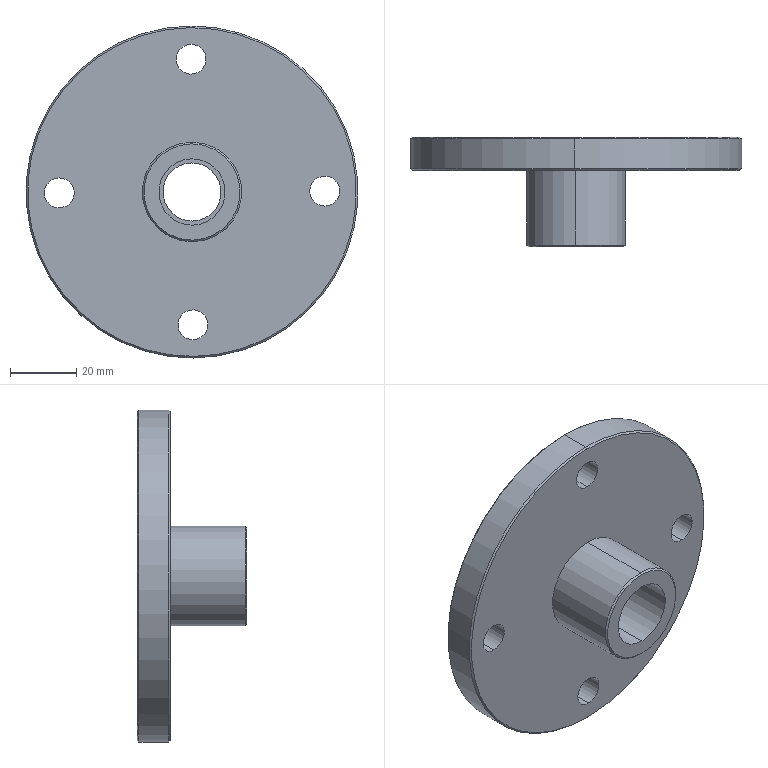Component | SolidWorks | E004Tray-1 | 1 solid | 28 faces | box 100 x 33 x 100 mm | volume 82304 mm3 | cylinder 16 | cone 8 | plane 4 | commonest cylinder face diameters 9 x8 20 x2 17.5 x2 100 x2 30 x2 | material Plain Carbon Steel
STEP:
#1=COLOUR_RGB('',0.7922,0.8196,0.9333);
#2=FILL_AREA_STYLE_COLOUR('',#1);
#3=FILL_AREA_STYLE('',(#2));
#4=SURFACE_STYLE_FILL_AREA(#3);
#5=SURFACE_SIDE_STYLE('',(#4));
#6=SURFACE_STYLE_USAGE(.BOTH.,#5);
#7=PRESENTATION_STYLE_ASSIGNMENT((#6));
#8=CARTESIAN_POINT('',(0.002756,9.764,-0.3937));
#9=VERTEX_POINT('',#8);
#10=CARTESIAN_POINT('',(-0.002756,9.764,0.3937));
#11=VERTEX_POINT('',#10);
#12=CARTESIAN_POINT('',(0.,9.764,0.));
#13=DIRECTION('',(0.,-1.,0.));
#14=DIRECTION('',(-0.006999,0.,1.));
#15=AXIS2_PLACEMENT_3D('',#12,#13,#14);
#16=CIRCLE('',#15,0.3937);
#17=EDGE_CURVE('',#9,#11,#16,.T.);
#18=ORIENTED_EDGE('',*,*,#17,.T.);
#19=CARTESIAN_POINT('',(-0.002756,10.787,0.3937));
#20=VERTEX_POINT('',#19);
#21=CARTESIAN_POINT('',(-0.002756,11.063,0.3937));
#22=DIRECTION('',(0.,1.,0.));
#23=VECTOR('',#22,39.37);
#24=LINE('',#21,#23);
#25=EDGE_CURVE('',#11,#20,#24,.T.);
#26=ORIENTED_EDGE('',*,*,#25,.T.);
#27=CARTESIAN_POINT('',(0.002756,10.787,-0.3937));
#28=VERTEX_POINT('',#27);
#29=CARTESIAN_POINT('',(0.,10.787,0.));
#30=DIRECTION('',(0.,1.,0.));
#31=DIRECTION('',(0.006999,0.,-1.));
#32=AXIS2_PLACEMENT_3D('',#29,#30,#31);
#33=CIRCLE('',#32,0.3937);
#34=EDGE_CURVE('',#20,#28,#33,.T.);
#35=ORIENTED_EDGE('',*,*,#34,.T.);
#36=CARTESIAN_POINT('',(0.002756,11.063,-0.3937));
#37=DIRECTION('',(0.,1.,0.));
#38=VECTOR('',#37,39.37);
#39=LINE('',#36,#38);
#40=EDGE_CURVE('',#9,#28,#39,.T.);
#41=ORIENTED_EDGE('',*,*,#40,.F.);
#42=EDGE_LOOP('',(#18,#26,#35,#41));
#43=FACE_OUTER_BOUND('',#42,.T.);
#44=CARTESIAN_POINT('',(0.,11.063,0.));
#45=DIRECTION('',(0.,1.,0.));
#46=DIRECTION('',(0.006999,0.,-1.));
#47=AXIS2_PLACEMENT_3D('',#44,#45,#46);
#48=CYLINDRICAL_SURFACE('',#47,0.3937);
#49=ADVANCED_FACE('',(#43),#48,.F.);
#50=CARTESIAN_POINT('',(-0.003996,9.764,0.5709));
#51=VERTEX_POINT('',#50);
#52=CARTESIAN_POINT('',(0.003996,9.764,-0.5709));
#53=VERTEX_POINT('',#52);
#54=CARTESIAN_POINT('',(0.,9.764,0.));
#55=DIRECTION('',(0.,-1.,0.));
#56=DIRECTION('',(-0.006999,0.,1.));
#57=AXIS2_PLACEMENT_3D('',#54,#55,#56);
#58=CIRCLE('',#57,0.5709);
#59=EDGE_CURVE('',#51,#53,#58,.T.);
#60=ORIENTED_EDGE('',*,*,#59,.F.);
#61=CARTESIAN_POINT('',(-0.004134,9.783,0.5905));
#62=VERTEX_POINT('',#61);
#63=CARTESIAN_POINT('',(-0.004134,9.783,0.5905));
#64=DIRECTION('',(-0.004949,0.7071,0.7071));
#65=VECTOR('',#64,39.37);
#66=LINE('',#63,#65);
#67=EDGE_CURVE('',#51,#62,#66,.T.);
#68=ORIENTED_EDGE('',*,*,#67,.T.);
#69=CARTESIAN_POINT('',(0.004134,9.783,-0.5905));
#70=VERTEX_POINT('',#69);
#71=CARTESIAN_POINT('',(0.,9.783,0.));
#72=DIRECTION('',(0.,1.,0.));
#73=DIRECTION('',(-0.006999,0.,1.));
#74=AXIS2_PLACEMENT_3D('',#71,#72,#73);
#75=CIRCLE('',#74,0.5906);
#76=EDGE_CURVE('',#70,#62,#75,.T.);
#77=ORIENTED_EDGE('',*,*,#76,.F.);
#78=CARTESIAN_POINT('',(0.004134,9.783,-0.5905));
#79=DIRECTION('',(0.004949,0.7071,-0.7071));
#80=VECTOR('',#79,39.37);
#81=LINE('',#78,#80);
#82=EDGE_CURVE('',#53,#70,#81,.T.);
#83=ORIENTED_EDGE('',*,*,#82,.F.);
#84=EDGE_LOOP('',(#60,#68,#77,#83));
#85=FACE_OUTER_BOUND('',#84,.T.);
#86=CARTESIAN_POINT('',(0.,9.783,0.));
#87=DIRECTION('',(0.,1.,0.));
#88=DIRECTION('',(0.006999,0.,-1.));
#89=AXIS2_PLACEMENT_3D('',#86,#87,#88);
#90=CONICAL_SURFACE('',#89,0.5906,0.7854);
#91=ADVANCED_FACE('',(#85),#90,.T.);
#92=CARTESIAN_POINT('',(-0.01364,10.669,1.949));
#93=VERTEX_POINT('',#92);
#94=CARTESIAN_POINT('',(0.01364,10.669,-1.949));
#95=VERTEX_POINT('',#94);
#96=CARTESIAN_POINT('',(0.,10.669,0.));
#97=DIRECTION('',(0.,-1.,0.));
#98=DIRECTION('',(-0.006999,0.,1.));
#99=AXIS2_PLACEMENT_3D('',#96,#97,#98);
#100=CIRCLE('',#99,1.949);
#101=EDGE_CURVE('',#93,#95,#100,.T.);
#102=ORIENTED_EDGE('',*,*,#101,.F.);
#103=CARTESIAN_POINT('',(-0.01378,10.689,1.968));
#104=VERTEX_POINT('',#103);
#105=CARTESIAN_POINT('',(-0.01378,10.689,1.968));
#106=DIRECTION('',(-0.004949,0.7071,0.7071));
#107=VECTOR('',#106,39.37);
#108=LINE('',#105,#107);
#109=EDGE_CURVE('',#93,#104,#108,.T.);
#110=ORIENTED_EDGE('',*,*,#109,.T.);
#111=CARTESIAN_POINT('',(0.01378,10.689,-1.968));
#112=VERTEX_POINT('',#111);
#113=CARTESIAN_POINT('',(0.,10.689,0.));
#114=DIRECTION('',(0.,1.,0.));
#115=DIRECTION('',(-0.006999,0.,1.));
#116=AXIS2_PLACEMENT_3D('',#113,#114,#115);
#117=CIRCLE('',#116,1.969);
#118=EDGE_CURVE('',#112,#104,#117,.T.);
#119=ORIENTED_EDGE('',*,*,#118,.F.);
#120=CARTESIAN_POINT('',(0.01378,10.689,-1.968));
#121=DIRECTION('',(0.004949,0.7071,-0.7071));
#122=VECTOR('',#121,39.37);
#123=LINE('',#120,#122);
#124=EDGE_CURVE('',#95,#112,#123,.T.);
#125=ORIENTED_EDGE('',*,*,#124,.F.);
#126=EDGE_LOOP('',(#102,#110,#119,#125));
#127=FACE_OUTER_BOUND('',#126,.T.);
#128=CARTESIAN_POINT('',(0.,10.689,0.));
#129=DIRECTION('',(0.,1.,0.));
#130=DIRECTION('',(0.006999,0.,-1.));
#131=AXIS2_PLACEMENT_3D('',#128,#129,#130);
#132=CONICAL_SURFACE('',#131,1.969,0.7854);
#133=ADVANCED_FACE('',(#127),#132,.T.);
#134=CARTESIAN_POINT('',(0.01364,11.063,-1.949));
#135=VERTEX_POINT('',#134);
#136=CARTESIAN_POINT('',(-0.01364,11.063,1.949));
#137=VERTEX_POINT('',#136);
#138=CARTESIAN_POINT('',(0.,11.063,0.));
#139=DIRECTION('',(0.,1.,0.));
#140=DIRECTION('',(0.006999,0.,-1.));
#141=AXIS2_PLACEMENT_3D('',#138,#139,#140);
#142=CIRCLE('',#141,1.949);
#143=EDGE_CURVE('',#135,#137,#142,.T.);
#144=ORIENTED_EDGE('',*,*,#143,.F.);
#145=CARTESIAN_POINT('',(0.01378,11.043,-1.968));
#146=VERTEX_POINT('',#145);
#147=CARTESIAN_POINT('',(0.01364,11.063,-1.949));
#148=DIRECTION('',(0.004949,-0.7071,-0.7071));
#149=VECTOR('',#148,39.37);
#150=LINE('',#147,#149);
#151=EDGE_CURVE('',#135,#146,#150,.T.);
#152=ORIENTED_EDGE('',*,*,#151,.T.);
#153=CARTESIAN_POINT('',(-0.01378,11.043,1.968));
#154=VERTEX_POINT('',#153);
#155=CARTESIAN_POINT('',(0.,11.043,0.));
#156=DIRECTION('',(0.,-1.,0.));
#157=DIRECTION('',(0.006999,0.,-1.));
#158=AXIS2_PLACEMENT_3D('',#155,#156,#157);
#159=CIRCLE('',#158,1.969);
#160=EDGE_CURVE('',#154,#146,#159,.T.);
#161=ORIENTED_EDGE('',*,*,#160,.F.);
#162=CARTESIAN_POINT('',(-0.01364,11.063,1.949));
#163=DIRECTION('',(-0.004949,-0.7071,0.7071));
#164=VECTOR('',#163,39.37);
#165=LINE('',#162,#164);
#166=EDGE_CURVE('',#137,#154,#165,.T.);
#167=ORIENTED_EDGE('',*,*,#166,.F.);
#168=EDGE_LOOP('',(#144,#152,#161,#167));
#169=FACE_OUTER_BOUND('',#168,.T.);
#170=CARTESIAN_POINT('',(0.,11.063,0.));
#171=DIRECTION('',(0.,-1.,0.));
#172=DIRECTION('',(-0.006999,0.,1.));
#173=AXIS2_PLACEMENT_3D('',#170,#171,#172);
#174=CONICAL_SURFACE('',#173,1.949,0.7854);
#175=ADVANCED_FACE('',(#169),#174,.T.);
#176=CARTESIAN_POINT('',(-0.002411,11.043,0.3445));
#177=VERTEX_POINT('',#176);
#178=CARTESIAN_POINT('',(0.002411,11.043,-0.3445));
#179=VERTEX_POINT('',#178);
#180=CARTESIAN_POINT('',(0.,11.043,0.));
#181=DIRECTION('',(0.,1.,0.));
#182=DIRECTION('',(0.006999,0.,-1.));
#183=AXIS2_PLACEMENT_3D('',#180,#181,#182);
#184=CIRCLE('',#183,0.3445);
#185=EDGE_CURVE('',#177,#179,#184,.T.);
#186=ORIENTED_EDGE('',*,*,#185,.F.);
#187=CARTESIAN_POINT('',(-0.002549,11.063,0.3642));
#188=VERTEX_POINT('',#187);
#189=CARTESIAN_POINT('',(-0.002411,11.043,0.3445));
#190=DIRECTION('',(-0.004949,0.7071,0.7071));
#191=VECTOR('',#190,39.37);
#192=LINE('',#189,#191);
#193=EDGE_CURVE('',#177,#188,#192,.T.);
#194=ORIENTED_EDGE('',*,*,#193,.T.);
#195=CARTESIAN_POINT('',(0.002549,11.063,-0.3642));
#196=VERTEX_POINT('',#195);
#197=CARTESIAN_POINT('',(0.,11.063,0.));
#198=DIRECTION('',(0.,-1.,0.));
#199=DIRECTION('',(0.006999,0.,-1.));
#200=AXIS2_PLACEMENT_3D('',#197,#198,#199);
#201=CIRCLE('',#200,0.3642);
#202=EDGE_CURVE('',#196,#188,#201,.T.);
#203=ORIENTED_EDGE('',*,*,#202,.F.);
#204=CARTESIAN_POINT('',(0.002411,11.043,-0.3445));
#205=DIRECTION('',(0.004949,0.7071,-0.7071));
#206=VECTOR('',#205,39.37);
#207=LINE('',#204,#206);
#208=EDGE_CURVE('',#179,#196,#207,.T.);
#209=ORIENTED_EDGE('',*,*,#208,.F.);
#210=EDGE_LOOP('',(#186,#194,#203,#209));
#211=FACE_OUTER_BOUND('',#210,.T.);
#212=CARTESIAN_POINT('',(0.,11.043,0.));
#213=DIRECTION('',(0.,1.,0.));
#214=DIRECTION('',(0.006999,0.,-1.));
#215=AXIS2_PLACEMENT_3D('',#212,#213,#214);
#216=CONICAL_SURFACE('',#215,0.3445,0.7854);
#217=ADVANCED_FACE('',(#211),#216,.F.);
#218=CARTESIAN_POINT('',(1.576,11.063,-0.1661));
#219=VERTEX_POINT('',#218);
#220=CARTESIAN_POINT('',(1.574,11.063,0.1882));
#221=VERTEX_POINT('',#220);
#222=CARTESIAN_POINT('',(1.575,11.063,0.01102));
#223=DIRECTION('',(0.,-1.,0.));
#224=DIRECTION('',(-1.,0.,-0.006999));
#225=AXIS2_PLACEMENT_3D('',#222,#223,#224);
#226=CIRCLE('',#225,0.1772);
#227=EDGE_CURVE('',#219,#221,#226,.T.);
#228=ORIENTED_EDGE('',*,*,#227,.F.);
#229=CARTESIAN_POINT('',(1.576,10.669,-0.1661));
#230=VERTEX_POINT('',#229);
#231=CARTESIAN_POINT('',(1.576,11.063,-0.1661));
#232=DIRECTION('',(0.,-1.,0.));
#233=VECTOR('',#232,39.37);
#234=LINE('',#231,#233);
#235=EDGE_CURVE('',#219,#230,#234,.T.);
#236=ORIENTED_EDGE('',*,*,#235,.T.);
#237=CARTESIAN_POINT('',(1.574,10.669,0.1882));
#238=VERTEX_POINT('',#237);
#239=CARTESIAN_POINT('',(1.575,10.669,0.01102));
#240=DIRECTION('',(0.,-1.,0.));
#241=DIRECTION('',(-1.,0.,-0.006999));
#242=AXIS2_PLACEMENT_3D('',#239,#240,#241);
#243=CIRCLE('',#242,0.1772);
#244=EDGE_CURVE('',#230,#238,#243,.T.);
#245=ORIENTED_EDGE('',*,*,#244,.T.);
#246=CARTESIAN_POINT('',(1.574,11.063,0.1882));
#247=DIRECTION('',(0.,-1.,0.));
#248=VECTOR('',#247,39.37);
#249=LINE('',#246,#248);
#250=EDGE_CURVE('',#221,#238,#249,.T.);
#251=ORIENTED_EDGE('',*,*,#250,.F.);
#252=EDGE_LOOP('',(#228,#236,#245,#251));
#253=FACE_OUTER_BOUND('',#252,.T.);
#254=CARTESIAN_POINT('',(1.575,11.063,0.01102));
#255=DIRECTION('',(0.,-1.,0.));
#256=DIRECTION('',(-0.006999,0.,1.));
#257=AXIS2_PLACEMENT_3D('',#254,#255,#256);
#258=CYLINDRICAL_SURFACE('',#257,0.1772);
#259=ADVANCED_FACE('',(#253),#258,.F.);
#260=CARTESIAN_POINT('',(-0.009783,11.063,1.398));
#261=VERTEX_POINT('',#260);
#262=CARTESIAN_POINT('',(-0.01226,11.063,1.752));
#263=VERTEX_POINT('',#262);
#264=CARTESIAN_POINT('',(-0.01102,11.063,1.575));
#265=DIRECTION('',(0.,-1.,0.));
#266=DIRECTION('',(0.006999,0.,-1.));
#267=AXIS2_PLACEMENT_3D('',#264,#265,#266);
#268=CIRCLE('',#267,0.1772);
#269=EDGE_CURVE('',#261,#263,#268,.T.);
#270=ORIENTED_EDGE('',*,*,#269,.F.);
#271=CARTESIAN_POINT('',(-0.009783,10.669,1.398));
#272=VERTEX_POINT('',#271);
#273=CARTESIAN_POINT('',(-0.009783,11.063,1.398));
#274=DIRECTION('',(0.,-1.,0.));
#275=VECTOR('',#274,39.37);
#276=LINE('',#273,#275);
#277=EDGE_CURVE('',#261,#272,#276,.T.);
#278=ORIENTED_EDGE('',*,*,#277,.T.);
#279=CARTESIAN_POINT('',(-0.01226,10.669,1.752));
#280=VERTEX_POINT('',#279);
#281=CARTESIAN_POINT('',(-0.01102,10.669,1.575));
#282=DIRECTION('',(0.,-1.,0.));
#283=DIRECTION('',(0.006999,0.,-1.));
#284=AXIS2_PLACEMENT_3D('',#281,#282,#283);
#285=CIRCLE('',#284,0.1772);
#286=EDGE_CURVE('',#272,#280,#285,.T.);
#287=ORIENTED_EDGE('',*,*,#286,.T.);
#288=CARTESIAN_POINT('',(-0.01226,11.063,1.752));
#289=DIRECTION('',(0.,-1.,0.));
#290=VECTOR('',#289,39.37);
#291=LINE('',#288,#290);
#292=EDGE_CURVE('',#263,#280,#291,.T.);
#293=ORIENTED_EDGE('',*,*,#292,.F.);
#294=EDGE_LOOP('',(#270,#278,#287,#293));
#295=FACE_OUTER_BOUND('',#294,.T.);
#296=CARTESIAN_POINT('',(-0.01102,11.063,1.575));
#297=DIRECTION('',(0.,-1.,0.));
#298=DIRECTION('',(-0.006999,0.,1.));
#299=AXIS2_PLACEMENT_3D('',#296,#297,#298);
#300=CYLINDRICAL_SURFACE('',#299,0.1772);
#301=ADVANCED_FACE('',(#295),#300,.F.);
#302=CARTESIAN_POINT('',(-1.574,11.063,-0.1882));
#303=VERTEX_POINT('',#302);
#304=CARTESIAN_POINT('',(-1.576,11.063,0.1661));
#305=VERTEX_POINT('',#304);
#306=CARTESIAN_POINT('',(-1.575,11.063,-0.01102));
#307=DIRECTION('',(0.,-1.,0.));
#308=DIRECTION('',(1.,0.,0.006999));
#309=AXIS2_PLACEMENT_3D('',#306,#307,#308);
#310=CIRCLE('',#309,0.1772);
#311=EDGE_CURVE('',#303,#305,#310,.T.);
#312=ORIENTED_EDGE('',*,*,#311,.F.);
#313=CARTESIAN_POINT('',(-1.574,10.669,-0.1882));
#314=VERTEX_POINT('',#313);
#315=CARTESIAN_POINT('',(-1.574,11.063,-0.1882));
#316=DIRECTION('',(0.,-1.,0.));
#317=VECTOR('',#316,39.37);
#318=LINE('',#315,#317);
#319=EDGE_CURVE('',#303,#314,#318,.T.);
#320=ORIENTED_EDGE('',*,*,#319,.T.);
#321=CARTESIAN_POINT('',(-1.576,10.669,0.1661));
#322=VERTEX_POINT('',#321);
#323=CARTESIAN_POINT('',(-1.575,10.669,-0.01102));
#324=DIRECTION('',(0.,-1.,0.));
#325=DIRECTION('',(1.,0.,0.006999));
#326=AXIS2_PLACEMENT_3D('',#323,#324,#325);
#327=CIRCLE('',#326,0.1772);
#328=EDGE_CURVE('',#314,#322,#327,.T.);
#329=ORIENTED_EDGE('',*,*,#328,.T.);
#330=CARTESIAN_POINT('',(-1.576,11.063,0.1661));
#331=DIRECTION('',(0.,-1.,0.));
#332=VECTOR('',#331,39.37);
#333=LINE('',#330,#332);
#334=EDGE_CURVE('',#305,#322,#333,.T.);
#335=ORIENTED_EDGE('',*,*,#334,.F.);
#336=EDGE_LOOP('',(#312,#320,#329,#335));
#337=FACE_OUTER_BOUND('',#336,.T.);
#338=CARTESIAN_POINT('',(-1.575,11.063,-0.01102));
#339=DIRECTION('',(0.,-1.,0.));
#340=DIRECTION('',(-0.006999,0.,1.));
#341=AXIS2_PLACEMENT_3D('',#338,#339,#340);
#342=CYLINDRICAL_SURFACE('',#341,0.1772);
#343=ADVANCED_FACE('',(#337),#342,.F.);
#344=CARTESIAN_POINT('',(0.01226,11.063,-1.752));
#345=VERTEX_POINT('',#344);
#346=CARTESIAN_POINT('',(0.009783,11.063,-1.398));
#347=VERTEX_POINT('',#346);
#348=CARTESIAN_POINT('',(0.01102,11.063,-1.575));
#349=DIRECTION('',(0.,-1.,0.));
#350=DIRECTION('',(-0.006999,0.,1.));
#351=AXIS2_PLACEMENT_3D('',#348,#349,#350);
#352=CIRCLE('',#351,0.1772);
#353=EDGE_CURVE('',#345,#347,#352,.T.);
#354=ORIENTED_EDGE('',*,*,#353,.F.);
#355=CARTESIAN_POINT('',(0.01226,10.669,-1.752));
#356=VERTEX_POINT('',#355);
#357=CARTESIAN_POINT('',(0.01226,11.063,-1.752));
#358=DIRECTION('',(0.,-1.,0.));
#359=VECTOR('',#358,39.37);
#360=LINE('',#357,#359);
#361=EDGE_CURVE('',#345,#356,#360,.T.);
#362=ORIENTED_EDGE('',*,*,#361,.T.);
#363=CARTESIAN_POINT('',(0.009783,10.669,-1.398));
#364=VERTEX_POINT('',#363);
#365=CARTESIAN_POINT('',(0.01102,10.669,-1.575));
#366=DIRECTION('',(0.,-1.,0.));
#367=DIRECTION('',(-0.006999,0.,1.));
#368=AXIS2_PLACEMENT_3D('',#365,#366,#367);
#369=CIRCLE('',#368,0.1772);
#370=EDGE_CURVE('',#356,#364,#369,.T.);
#371=ORIENTED_EDGE('',*,*,#370,.T.);
#372=CARTESIAN_POINT('',(0.009783,11.063,-1.398));
#373=DIRECTION('',(0.,-1.,0.));
#374=VECTOR('',#373,39.37);
#375=LINE('',#372,#374);
#376=EDGE_CURVE('',#347,#364,#375,.T.);
#377=ORIENTED_EDGE('',*,*,#376,.F.);
#378=EDGE_LOOP('',(#354,#362,#371,#377));
#379=FACE_OUTER_BOUND('',#378,.T.);
#380=CARTESIAN_POINT('',(0.01102,11.063,-1.575));
#381=DIRECTION('',(0.,-1.,0.));
#382=DIRECTION('',(-0.006999,0.,1.));
#383=AXIS2_PLACEMENT_3D('',#380,#381,#382);
#384=CYLINDRICAL_SURFACE('',#383,0.1772);
#385=ADVANCED_FACE('',(#379),#384,.F.);
#386=ORIENTED_EDGE('',*,*,#185,.T.);
#387=CARTESIAN_POINT('',(0.002411,10.787,-0.3445));
#388=VERTEX_POINT('',#387);
#389=CARTESIAN_POINT('',(0.002411,9.764,-0.3445));
#390=DIRECTION('',(0.,-1.,0.));
#391=VECTOR('',#390,39.37);
#392=LINE('',#389,#391);
#393=EDGE_CURVE('',#179,#388,#392,.T.);
#394=ORIENTED_EDGE('',*,*,#393,.T.);
#395=CARTESIAN_POINT('',(-0.002411,10.787,0.3445));
#396=VERTEX_POINT('',#395);
#397=CARTESIAN_POINT('',(0.,10.787,0.));
#398=DIRECTION('',(0.,-1.,0.));
#399=DIRECTION('',(0.006999,0.,-1.));
#400=AXIS2_PLACEMENT_3D('',#397,#398,#399);
#401=CIRCLE('',#400,0.3445);
#402=EDGE_CURVE('',#388,#396,#401,.T.);
#403=ORIENTED_EDGE('',*,*,#402,.T.);
#404=CARTESIAN_POINT('',(-0.002411,9.764,0.3445));
#405=DIRECTION('',(0.,-1.,0.));
#406=VECTOR('',#405,39.37);
#407=LINE('',#404,#406);
#408=EDGE_CURVE('',#177,#396,#407,.T.);
#409=ORIENTED_EDGE('',*,*,#408,.F.);
#410=EDGE_LOOP('',(#386,#394,#403,#409));
#411=FACE_OUTER_BOUND('',#410,.T.);
#412=CARTESIAN_POINT('',(0.,9.764,0.));
#413=DIRECTION('',(0.,-1.,0.));
#414=DIRECTION('',(-0.006999,0.,1.));
#415=AXIS2_PLACEMENT_3D('',#412,#413,#414);
#416=CYLINDRICAL_SURFACE('',#415,0.3445);
#417=ADVANCED_FACE('',(#411),#416,.F.);
#418=ORIENTED_EDGE('',*,*,#118,.T.);
#419=CARTESIAN_POINT('',(-0.01378,11.063,1.968));
#420=DIRECTION('',(0.,1.,0.));
#421=VECTOR('',#420,39.37);
#422=LINE('',#419,#421);
#423=EDGE_CURVE('',#104,#154,#422,.T.);
#424=ORIENTED_EDGE('',*,*,#423,.T.);
#425=ORIENTED_EDGE('',*,*,#160,.T.);
#426=CARTESIAN_POINT('',(0.01378,11.063,-1.968));
#427=DIRECTION('',(0.,1.,0.));
#428=VECTOR('',#427,39.37);
#429=LINE('',#426,#428);
#430=EDGE_CURVE('',#112,#146,#429,.T.);
#431=ORIENTED_EDGE('',*,*,#430,.F.);
#432=EDGE_LOOP('',(#418,#424,#425,#431));
#433=FACE_OUTER_BOUND('',#432,.T.);
#434=CARTESIAN_POINT('',(0.,11.063,0.));
#435=DIRECTION('',(0.,1.,0.));
#436=DIRECTION('',(0.006999,0.,-1.));
#437=AXIS2_PLACEMENT_3D('',#434,#435,#436);
#438=CYLINDRICAL_SURFACE('',#437,1.969);
#439=ADVANCED_FACE('',(#433),#438,.T.);
#440=ORIENTED_EDGE('',*,*,#76,.T.);
#441=CARTESIAN_POINT('',(-0.004134,10.669,0.5905));
#442=VERTEX_POINT('',#441);
#443=CARTESIAN_POINT('',(-0.004134,11.063,0.5905));
#444=DIRECTION('',(0.,1.,0.));
#445=VECTOR('',#444,39.37);
#446=LINE('',#443,#445);
#447=EDGE_CURVE('',#62,#442,#446,.T.);
#448=ORIENTED_EDGE('',*,*,#447,.T.);
#449=CARTESIAN_POINT('',(0.004134,10.669,-0.5905));
#450=VERTEX_POINT('',#449);
#451=CARTESIAN_POINT('',(0.,10.669,0.));
#452=DIRECTION('',(0.,1.,0.));
#453=DIRECTION('',(0.006999,0.,-1.));
#454=AXIS2_PLACEMENT_3D('',#451,#452,#453);
#455=CIRCLE('',#454,0.5906);
#456=EDGE_CURVE('',#450,#442,#455,.T.);
#457=ORIENTED_EDGE('',*,*,#456,.F.);
#458=CARTESIAN_POINT('',(0.004134,11.063,-0.5905));
#459=DIRECTION('',(0.,1.,0.));
#460=VECTOR('',#459,39.37);
#461=LINE('',#458,#460);
#462=EDGE_CURVE('',#70,#450,#461,.T.);
#463=ORIENTED_EDGE('',*,*,#462,.F.);
#464=EDGE_LOOP('',(#440,#448,#457,#463));
#465=FACE_OUTER_BOUND('',#464,.T.);
#466=CARTESIAN_POINT('',(0.,11.063,0.));
#467=DIRECTION('',(0.,1.,0.));
#468=DIRECTION('',(0.006999,0.,-1.));
#469=AXIS2_PLACEMENT_3D('',#466,#467,#468);
#470=CYLINDRICAL_SURFACE('',#469,0.5906);
#471=ADVANCED_FACE('',(#465),#470,.T.);
#472=ORIENTED_EDGE('',*,*,#17,.F.);
#473=CARTESIAN_POINT('',(0.,9.764,0.));
#474=DIRECTION('',(0.,-1.,0.));
#475=DIRECTION('',(-0.006999,0.,1.));
#476=AXIS2_PLACEMENT_3D('',#473,#474,#475);
#477=CIRCLE('',#476,0.3937);
#478=EDGE_CURVE('',#11,#9,#477,.T.);
#479=ORIENTED_EDGE('',*,*,#478,.F.);
#480=EDGE_LOOP('',(#472,#479));
#481=FACE_BOUND('',#480,.T.);
#482=CARTESIAN_POINT('',(0.,9.764,0.));
#483=DIRECTION('',(0.,-1.,0.));
#484=DIRECTION('',(-0.006999,0.,1.));
#485=AXIS2_PLACEMENT_3D('',#482,#483,#484);
#486=CIRCLE('',#485,0.5709);
#487=EDGE_CURVE('',#53,#51,#486,.T.);
#488=ORIENTED_EDGE('',*,*,#487,.T.);
#489=ORIENTED_EDGE('',*,*,#59,.T.);
#490=EDGE_LOOP('',(#488,#489));
#491=FACE_OUTER_BOUND('',#490,.T.);
#492=CARTESIAN_POINT('',(0.,9.764,0.));
#493=DIRECTION('',(0.,-1.,0.));
#494=DIRECTION('',(-0.006999,0.,1.));
#495=AXIS2_PLACEMENT_3D('',#492,#493,#494);
#496=PLANE('',#495);
#497=ADVANCED_FACE('',(#481,#491),#496,.T.);
#498=ORIENTED_EDGE('',*,*,#447,.F.);
#499=CARTESIAN_POINT('',(0.,9.783,0.));
#500=DIRECTION('',(0.,1.,0.));
#501=DIRECTION('',(-0.006999,0.,1.));
#502=AXIS2_PLACEMENT_3D('',#499,#500,#501);
#503=CIRCLE('',#502,0.5906);
#504=EDGE_CURVE('',#62,#70,#503,.T.);
#505=ORIENTED_EDGE('',*,*,#504,.T.);
#506=ORIENTED_EDGE('',*,*,#462,.T.);
#507=CARTESIAN_POINT('',(0.,10.669,0.));
#508=DIRECTION('',(0.,1.,0.));
#509=DIRECTION('',(0.006999,0.,-1.));
#510=AXIS2_PLACEMENT_3D('',#507,#508,#509);
#511=CIRCLE('',#510,0.5906);
#512=EDGE_CURVE('',#442,#450,#511,.T.);
#513=ORIENTED_EDGE('',*,*,#512,.F.);
#514=EDGE_LOOP('',(#498,#505,#506,#513));
#515=FACE_OUTER_BOUND('',#514,.T.);
#516=CARTESIAN_POINT('',(0.,11.063,0.));
#517=DIRECTION('',(0.,1.,0.));
#518=DIRECTION('',(0.006999,0.,-1.));
#519=AXIS2_PLACEMENT_3D('',#516,#517,#518);
#520=CYLINDRICAL_SURFACE('',#519,0.5906);
#521=ADVANCED_FACE('',(#515),#520,.T.);
#522=CARTESIAN_POINT('',(0.,10.669,0.));
#523=DIRECTION('',(0.,-1.,0.));
#524=DIRECTION('',(-0.006999,0.,1.));
#525=AXIS2_PLACEMENT_3D('',#522,#523,#524);
#526=CIRCLE('',#525,1.949);
#527=EDGE_CURVE('',#95,#93,#526,.T.);
#528=ORIENTED_EDGE('',*,*,#527,.T.);
#529=ORIENTED_EDGE('',*,*,#101,.T.);
#530=EDGE_LOOP('',(#528,#529));
#531=FACE_OUTER_BOUND('',#530,.T.);
#532=CARTESIAN_POINT('',(1.575,10.669,0.01102));
#533=DIRECTION('',(0.,-1.,0.));
#534=DIRECTION('',(-1.,0.,-0.006999));
#535=AXIS2_PLACEMENT_3D('',#532,#533,#534);
#536=CIRCLE('',#535,0.1772);
#537=EDGE_CURVE('',#238,#230,#536,.T.);
#538=ORIENTED_EDGE('',*,*,#537,.F.);
#539=ORIENTED_EDGE('',*,*,#244,.F.);
#540=EDGE_LOOP('',(#538,#539));
#541=FACE_BOUND('',#540,.T.);
#542=CARTESIAN_POINT('',(-0.01102,10.669,1.575));
#543=DIRECTION('',(0.,-1.,0.));
#544=DIRECTION('',(0.006999,0.,-1.));
#545=AXIS2_PLACEMENT_3D('',#542,#543,#544);
#546=CIRCLE('',#545,0.1772);
#547=EDGE_CURVE('',#280,#272,#546,.T.);
#548=ORIENTED_EDGE('',*,*,#547,.F.);
#549=ORIENTED_EDGE('',*,*,#286,.F.);
#550=EDGE_LOOP('',(#548,#549));
#551=FACE_BOUND('',#550,.T.);
#552=CARTESIAN_POINT('',(-1.575,10.669,-0.01102));
#553=DIRECTION('',(0.,-1.,0.));
#554=DIRECTION('',(1.,0.,0.006999));
#555=AXIS2_PLACEMENT_3D('',#552,#553,#554);
#556=CIRCLE('',#555,0.1772);
#557=EDGE_CURVE('',#322,#314,#556,.T.);
#558=ORIENTED_EDGE('',*,*,#557,.F.);
#559=ORIENTED_EDGE('',*,*,#328,.F.);
#560=EDGE_LOOP('',(#558,#559));
#561=FACE_BOUND('',#560,.T.);
#562=CARTESIAN_POINT('',(0.01102,10.669,-1.575));
#563=DIRECTION('',(0.,-1.,0.));
#564=DIRECTION('',(-0.006999,0.,1.));
#565=AXIS2_PLACEMENT_3D('',#562,#563,#564);
#566=CIRCLE('',#565,0.1772);
#567=EDGE_CURVE('',#364,#356,#566,.T.);
#568=ORIENTED_EDGE('',*,*,#567,.F.);
#569=ORIENTED_EDGE('',*,*,#370,.F.);
#570=EDGE_LOOP('',(#568,#569));
#571=FACE_BOUND('',#570,.T.);
#572=ORIENTED_EDGE('',*,*,#456,.T.);
#573=ORIENTED_EDGE('',*,*,#512,.T.);
#574=EDGE_LOOP('',(#572,#573));
#575=FACE_BOUND('',#574,.T.);
#576=CARTESIAN_POINT('',(-0.5905,10.669,-0.004134));
#577=DIRECTION('',(0.,-1.,0.));
#578=DIRECTION('',(-0.006999,0.,1.));
#579=AXIS2_PLACEMENT_3D('',#576,#577,#578);
#580=PLANE('',#579);
#581=ADVANCED_FACE('',(#531,#541,#551,#561,#571,#575),#580,.T.);
#582=ORIENTED_EDGE('',*,*,#423,.F.);
#583=CARTESIAN_POINT('',(0.,10.689,0.));
#584=DIRECTION('',(0.,1.,0.));
#585=DIRECTION('',(-0.006999,0.,1.));
#586=AXIS2_PLACEMENT_3D('',#583,#584,#585);
#587=CIRCLE('',#586,1.969);
#588=EDGE_CURVE('',#104,#112,#587,.T.);
#589=ORIENTED_EDGE('',*,*,#588,.T.);
#590=ORIENTED_EDGE('',*,*,#430,.T.);
#591=CARTESIAN_POINT('',(0.,11.043,0.));
#592=DIRECTION('',(0.,-1.,0.));
#593=DIRECTION('',(0.006999,0.,-1.));
#594=AXIS2_PLACEMENT_3D('',#591,#592,#593);
#595=CIRCLE('',#594,1.969);
#596=EDGE_CURVE('',#146,#154,#595,.T.);
#597=ORIENTED_EDGE('',*,*,#596,.T.);
#598=EDGE_LOOP('',(#582,#589,#590,#597));
#599=FACE_OUTER_BOUND('',#598,.T.);
#600=CARTESIAN_POINT('',(0.,11.063,0.));
#601=DIRECTION('',(0.,1.,0.));
#602=DIRECTION('',(0.006999,0.,-1.));
#603=AXIS2_PLACEMENT_3D('',#600,#601,#602);
#604=CYLINDRICAL_SURFACE('',#603,1.969);
#605=ADVANCED_FACE('',(#599),#604,.T.);
#606=ORIENTED_EDGE('',*,*,#202,.T.);
#607=CARTESIAN_POINT('',(0.,11.063,0.));
#608=DIRECTION('',(0.,-1.,0.));
#609=DIRECTION('',(0.006999,0.,-1.));
#610=AXIS2_PLACEMENT_3D('',#607,#608,#609);
#611=CIRCLE('',#610,0.3642);
#612=EDGE_CURVE('',#188,#196,#611,.T.);
#613=ORIENTED_EDGE('',*,*,#612,.T.);
#614=EDGE_LOOP('',(#606,#613));
#615=FACE_BOUND('',#614,.T.);
#616=CARTESIAN_POINT('',(0.,11.063,0.));
#617=DIRECTION('',(0.,1.,0.));
#618=DIRECTION('',(0.006999,0.,-1.));
#619=AXIS2_PLACEMENT_3D('',#616,#617,#618);
#620=CIRCLE('',#619,1.949);
#621=EDGE_CURVE('',#137,#135,#620,.T.);
#622=ORIENTED_EDGE('',*,*,#621,.T.);
#623=ORIENTED_EDGE('',*,*,#143,.T.);
#624=EDGE_LOOP('',(#622,#623));
#625=FACE_OUTER_BOUND('',#624,.T.);
#626=CARTESIAN_POINT('',(1.575,11.063,0.01102));
#627=DIRECTION('',(0.,-1.,0.));
#628=DIRECTION('',(-1.,0.,-0.006999));
#629=AXIS2_PLACEMENT_3D('',#626,#627,#628);
#630=CIRCLE('',#629,0.1772);
#631=EDGE_CURVE('',#221,#219,#630,.T.);
#632=ORIENTED_EDGE('',*,*,#631,.T.);
#633=ORIENTED_EDGE('',*,*,#227,.T.);
#634=EDGE_LOOP('',(#632,#633));
#635=FACE_BOUND('',#634,.T.);
#636=CARTESIAN_POINT('',(-0.01102,11.063,1.575));
#637=DIRECTION('',(0.,-1.,0.));
#638=DIRECTION('',(0.006999,0.,-1.));
#639=AXIS2_PLACEMENT_3D('',#636,#637,#638);
#640=CIRCLE('',#639,0.1772);
#641=EDGE_CURVE('',#263,#261,#640,.T.);
#642=ORIENTED_EDGE('',*,*,#641,.T.);
#643=ORIENTED_EDGE('',*,*,#269,.T.);
#644=EDGE_LOOP('',(#642,#643));
#645=FACE_BOUND('',#644,.T.);
#646=CARTESIAN_POINT('',(-1.575,11.063,-0.01102));
#647=DIRECTION('',(0.,-1.,0.));
#648=DIRECTION('',(1.,0.,0.006999));
#649=AXIS2_PLACEMENT_3D('',#646,#647,#648);
#650=CIRCLE('',#649,0.1772);
#651=EDGE_CURVE('',#305,#303,#650,.T.);
#652=ORIENTED_EDGE('',*,*,#651,.T.);
#653=ORIENTED_EDGE('',*,*,#311,.T.);
#654=EDGE_LOOP('',(#652,#653));
#655=FACE_BOUND('',#654,.T.);
#656=CARTESIAN_POINT('',(0.01102,11.063,-1.575));
#657=DIRECTION('',(0.,-1.,0.));
#658=DIRECTION('',(-0.006999,0.,1.));
#659=AXIS2_PLACEMENT_3D('',#656,#657,#658);
#660=CIRCLE('',#659,0.1772);
#661=EDGE_CURVE('',#347,#345,#660,.T.);
#662=ORIENTED_EDGE('',*,*,#661,.T.);
#663=ORIENTED_EDGE('',*,*,#353,.T.);
#664=EDGE_LOOP('',(#662,#663));
#665=FACE_BOUND('',#664,.T.);
#666=CARTESIAN_POINT('',(-1.968,11.063,-0.01378));
#667=DIRECTION('',(0.,1.,0.));
#668=DIRECTION('',(0.006999,0.,-1.));
#669=AXIS2_PLACEMENT_3D('',#666,#667,#668);
#670=PLANE('',#669);
#671=ADVANCED_FACE('',(#615,#625,#635,#645,#655,#665),#670,.T.);
#672=ORIENTED_EDGE('',*,*,#393,.F.);
#673=CARTESIAN_POINT('',(0.,11.043,0.));
#674=DIRECTION('',(0.,1.,0.));
#675=DIRECTION('',(0.006999,0.,-1.));
#676=AXIS2_PLACEMENT_3D('',#673,#674,#675);
#677=CIRCLE('',#676,0.3445);
#678=EDGE_CURVE('',#179,#177,#677,.T.);
#679=ORIENTED_EDGE('',*,*,#678,.T.);
#680=ORIENTED_EDGE('',*,*,#408,.T.);
#681=CARTESIAN_POINT('',(0.,10.787,0.));
#682=DIRECTION('',(0.,-1.,0.));
#683=DIRECTION('',(0.006999,0.,-1.));
#684=AXIS2_PLACEMENT_3D('',#681,#682,#683);
#685=CIRCLE('',#684,0.3445);
#686=EDGE_CURVE('',#396,#388,#685,.T.);
#687=ORIENTED_EDGE('',*,*,#686,.T.);
#688=EDGE_LOOP('',(#672,#679,#680,#687));
#689=FACE_OUTER_BOUND('',#688,.T.);
#690=CARTESIAN_POINT('',(0.,9.764,0.));
#691=DIRECTION('',(0.,-1.,0.));
#692=DIRECTION('',(-0.006999,0.,1.));
#693=AXIS2_PLACEMENT_3D('',#690,#691,#692);
#694=CYLINDRICAL_SURFACE('',#693,0.3445);
#695=ADVANCED_FACE('',(#689),#694,.F.);
#696=ORIENTED_EDGE('',*,*,#361,.F.);
#697=ORIENTED_EDGE('',*,*,#661,.F.);
#698=ORIENTED_EDGE('',*,*,#376,.T.);
#699=ORIENTED_EDGE('',*,*,#567,.T.);
#700=EDGE_LOOP('',(#696,#697,#698,#699));
#701=FACE_OUTER_BOUND('',#700,.T.);
#702=CARTESIAN_POINT('',(0.01102,11.063,-1.575));
#703=DIRECTION('',(0.,-1.,0.));
#704=DIRECTION('',(-0.006999,0.,1.));
#705=AXIS2_PLACEMENT_3D('',#702,#703,#704);
#706=CYLINDRICAL_SURFACE('',#705,0.1772);
#707=ADVANCED_FACE('',(#701),#706,.F.);
#708=ORIENTED_EDGE('',*,*,#319,.F.);
#709=ORIENTED_EDGE('',*,*,#651,.F.);
#710=ORIENTED_EDGE('',*,*,#334,.T.);
#711=ORIENTED_EDGE('',*,*,#557,.T.);
#712=EDGE_LOOP('',(#708,#709,#710,#711));
#713=FACE_OUTER_BOUND('',#712,.T.);
#714=CARTESIAN_POINT('',(-1.575,11.063,-0.01102));
#715=DIRECTION('',(0.,-1.,0.));
#716=DIRECTION('',(-0.006999,0.,1.));
#717=AXIS2_PLACEMENT_3D('',#714,#715,#716);
#718=CYLINDRICAL_SURFACE('',#717,0.1772);
#719=ADVANCED_FACE('',(#713),#718,.F.);
#720=ORIENTED_EDGE('',*,*,#277,.F.);
#721=ORIENTED_EDGE('',*,*,#641,.F.);
#722=ORIENTED_EDGE('',*,*,#292,.T.);
#723=ORIENTED_EDGE('',*,*,#547,.T.);
#724=EDGE_LOOP('',(#720,#721,#722,#723));
#725=FACE_OUTER_BOUND('',#724,.T.);
#726=CARTESIAN_POINT('',(-0.01102,11.063,1.575));
#727=DIRECTION('',(0.,-1.,0.));
#728=DIRECTION('',(-0.006999,0.,1.));
#729=AXIS2_PLACEMENT_3D('',#726,#727,#728);
#730=CYLINDRICAL_SURFACE('',#729,0.1772);
#731=ADVANCED_FACE('',(#725),#730,.F.);
#732=ORIENTED_EDGE('',*,*,#235,.F.);
#733=ORIENTED_EDGE('',*,*,#631,.F.);
#734=ORIENTED_EDGE('',*,*,#250,.T.);
#735=ORIENTED_EDGE('',*,*,#537,.T.);
#736=EDGE_LOOP('',(#732,#733,#734,#735));
#737=FACE_OUTER_BOUND('',#736,.T.);
#738=CARTESIAN_POINT('',(1.575,11.063,0.01102));
#739=DIRECTION('',(0.,-1.,0.));
#740=DIRECTION('',(-0.006999,0.,1.));
#741=AXIS2_PLACEMENT_3D('',#738,#739,#740);
#742=CYLINDRICAL_SURFACE('',#741,0.1772);
#743=ADVANCED_FACE('',(#737),#742,.F.);
#744=ORIENTED_EDGE('',*,*,#193,.F.);
#745=ORIENTED_EDGE('',*,*,#678,.F.);
#746=ORIENTED_EDGE('',*,*,#208,.T.);
#747=ORIENTED_EDGE('',*,*,#612,.F.);
#748=EDGE_LOOP('',(#744,#745,#746,#747));
#749=FACE_OUTER_BOUND('',#748,.T.);
#750=CARTESIAN_POINT('',(0.,11.043,0.));
#751=DIRECTION('',(0.,1.,0.));
#752=DIRECTION('',(0.006999,0.,-1.));
#753=AXIS2_PLACEMENT_3D('',#750,#751,#752);
#754=CONICAL_SURFACE('',#753,0.3445,0.7854);
#755=ADVANCED_FACE('',(#749),#754,.F.);
#756=ORIENTED_EDGE('',*,*,#151,.F.);
#757=ORIENTED_EDGE('',*,*,#621,.F.);
#758=ORIENTED_EDGE('',*,*,#166,.T.);
#759=ORIENTED_EDGE('',*,*,#596,.F.);
#760=EDGE_LOOP('',(#756,#757,#758,#759));
#761=FACE_OUTER_BOUND('',#760,.T.);
#762=CARTESIAN_POINT('',(0.,11.063,0.));
#763=DIRECTION('',(0.,-1.,0.));
#764=DIRECTION('',(-0.006999,0.,1.));
#765=AXIS2_PLACEMENT_3D('',#762,#763,#764);
#766=CONICAL_SURFACE('',#765,1.949,0.7854);
#767=ADVANCED_FACE('',(#761),#766,.T.);
#768=ORIENTED_EDGE('',*,*,#109,.F.);
#769=ORIENTED_EDGE('',*,*,#527,.F.);
#770=ORIENTED_EDGE('',*,*,#124,.T.);
#771=ORIENTED_EDGE('',*,*,#588,.F.);
#772=EDGE_LOOP('',(#768,#769,#770,#771));
#773=FACE_OUTER_BOUND('',#772,.T.);
#774=CARTESIAN_POINT('',(0.,10.689,0.));
#775=DIRECTION('',(0.,1.,0.));
#776=DIRECTION('',(0.006999,0.,-1.));
#777=AXIS2_PLACEMENT_3D('',#774,#775,#776);
#778=CONICAL_SURFACE('',#777,1.969,0.7854);
#779=ADVANCED_FACE('',(#773),#778,.T.);
#780=ORIENTED_EDGE('',*,*,#67,.F.);
#781=ORIENTED_EDGE('',*,*,#487,.F.);
#782=ORIENTED_EDGE('',*,*,#82,.T.);
#783=ORIENTED_EDGE('',*,*,#504,.F.);
#784=EDGE_LOOP('',(#780,#781,#782,#783));
#785=FACE_OUTER_BOUND('',#784,.T.);
#786=CARTESIAN_POINT('',(0.,9.783,0.));
#787=DIRECTION('',(0.,1.,0.));
#788=DIRECTION('',(0.006999,0.,-1.));
#789=AXIS2_PLACEMENT_3D('',#786,#787,#788);
#790=CONICAL_SURFACE('',#789,0.5906,0.7854);
#791=ADVANCED_FACE('',(#785),#790,.T.);
#792=CARTESIAN_POINT('',(0.,10.787,0.));
#793=DIRECTION('',(0.,1.,0.));
#794=DIRECTION('',(0.006999,0.,-1.));
#795=AXIS2_PLACEMENT_3D('',#792,#793,#794);
#796=CIRCLE('',#795,0.3937);
#797=EDGE_CURVE('',#28,#20,#796,.T.);
#798=ORIENTED_EDGE('',*,*,#797,.F.);
#799=ORIENTED_EDGE('',*,*,#34,.F.);
#800=EDGE_LOOP('',(#798,#799));
#801=FACE_OUTER_BOUND('',#800,.T.);
#802=ORIENTED_EDGE('',*,*,#686,.F.);
#803=ORIENTED_EDGE('',*,*,#402,.F.);
#804=EDGE_LOOP('',(#802,#803));
#805=FACE_BOUND('',#804,.T.);
#806=CARTESIAN_POINT('',(0.,10.787,0.));
#807=DIRECTION('',(0.,1.,0.));
#808=DIRECTION('',(0.006999,0.,-1.));
#809=AXIS2_PLACEMENT_3D('',#806,#807,#808);
#810=PLANE('',#809);
#811=ADVANCED_FACE('',(#801,#805),#810,.F.);
#812=ORIENTED_EDGE('',*,*,#25,.F.);
#813=ORIENTED_EDGE('',*,*,#478,.T.);
#814=ORIENTED_EDGE('',*,*,#40,.T.);
#815=ORIENTED_EDGE('',*,*,#797,.T.);
#816=EDGE_LOOP('',(#812,#813,#814,#815));
#817=FACE_OUTER_BOUND('',#816,.T.);
#818=CARTESIAN_POINT('',(0.,11.063,0.));
#819=DIRECTION('',(0.,1.,0.));
#820=DIRECTION('',(0.006999,0.,-1.));
#821=AXIS2_PLACEMENT_3D('',#818,#819,#820);
#822=CYLINDRICAL_SURFACE('',#821,0.3937);
#823=ADVANCED_FACE('',(#817),#822,.F.);
#824=CLOSED_SHELL('',(#49,#91,#133,#175,#217,#259,#301,#343,#385,#417,#439,#471,#497,#521,#581,#605,#671,#695,#707,#719,#731,#743,#755,#767,#779,#791,#811,#823));
#825=MANIFOLD_SOLID_BREP('',#824);
#826=STYLED_ITEM('',(#7),#825);
#827=(LENGTH_UNIT()NAMED_UNIT(*)SI_UNIT($,.METRE.));
#828=LENGTH_MEASURE_WITH_UNIT(LENGTH_MEASURE(0.0254),#827);
#829=DIMENSIONAL_EXPONENTS(1.,0.,0.,0.,0.,0.,0.);
#830=(CONVERSION_BASED_UNIT('',#828)LENGTH_UNIT()NAMED_UNIT(#829));
#831=UNCERTAINTY_MEASURE_WITH_UNIT(LENGTH_MEASURE(0.00001),#830,'','');
#832=(NAMED_UNIT(*)PLANE_ANGLE_UNIT()SI_UNIT($,.RADIAN.));
#833=(NAMED_UNIT(*)SI_UNIT($,.STERADIAN.)SOLID_ANGLE_UNIT());
#834=(GEOMETRIC_REPRESENTATION_CONTEXT(3)GLOBAL_UNCERTAINTY_ASSIGNED_CONTEXT((#831))GLOBAL_UNIT_ASSIGNED_CONTEXT((#830,#832,#833))REPRESENTATION_CONTEXT('',''));
#835=MECHANICAL_DESIGN_GEOMETRIC_PRESENTATION_REPRESENTATION('',(#826),#834);
#836=PRESENTATION_LAYER_ASSIGNMENT('','',(#826));
#837=CARTESIAN_POINT('',(0.,0.,0.));
#838=DIRECTION('',(0.,0.,1.));
#839=DIRECTION('',(1.,0.,0.));
#840=AXIS2_PLACEMENT_3D('',#837,#838,#839);
#841=(LENGTH_UNIT()NAMED_UNIT(*)SI_UNIT($,.METRE.));
#842=LENGTH_MEASURE_WITH_UNIT(LENGTH_MEASURE(0.0254),#841);
#843=DIMENSIONAL_EXPONENTS(1.,0.,0.,0.,0.,0.,0.);
#844=(CONVERSION_BASED_UNIT('',#842)LENGTH_UNIT()NAMED_UNIT(#843));
#845=UNCERTAINTY_MEASURE_WITH_UNIT(LENGTH_MEASURE(0.00001),#844,'','');
#846=(NAMED_UNIT(*)PLANE_ANGLE_UNIT()SI_UNIT($,.RADIAN.));
#847=(NAMED_UNIT(*)SI_UNIT($,.STERADIAN.)SOLID_ANGLE_UNIT());
#848=(GEOMETRIC_REPRESENTATION_CONTEXT(3)GLOBAL_UNCERTAINTY_ASSIGNED_CONTEXT((#845))GLOBAL_UNIT_ASSIGNED_CONTEXT((#844,#846,#847))REPRESENTATION_CONTEXT('',''));
#849=ADVANCED_BREP_SHAPE_REPRESENTATION('',(#825,#840),#848);